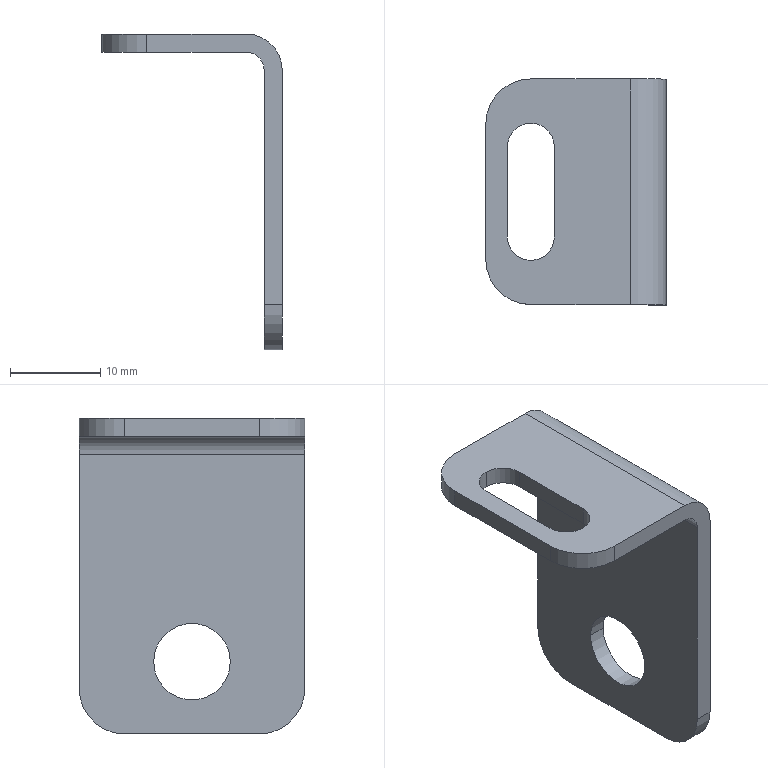Component | SolidWorks | YX-04-119GlueFeedingProximitySwitchFixingPlate-1 | 1 solid | 21 faces | box 20 x 25 x 35 mm | volume 2283 mm3 | cylinder 11 | plane 10 | commonest cylinder face diameters 10 x4 5.2 x3 8.5 x2 4 x1 8 x1 | material SUS340
build123d program:
from build123d import *

# Parameters (mm, degrees)
SKETCH1_W                      = 35
SKETCH1_H                      = 25
BOSS_EXTRUDE1_DEPTH            = 20
SKETCH2_W                      = 33
SKETCH2_H                      = 18
CUT_EXTRUDE1_DEPTH             = 48.434
CUT_EXTRUDE2_DEPTH             = 43.205
F_8_5_8_5_DIAMETER_HOLE1_D     = 8.5
F_8_5_8_5_DIAMETER_HOLE1_DEPTH = 20
FILLET1_R                      = 2
FILLET2_R                      = 4
FILLET3_R                      = 5


with BuildPart() as part:
    # Sketch1 → Boss-Extrude1 (new body)
    with BuildSketch(Plane(origin=(0, 20, 0), x_dir=(1, 0, 0), z_dir=(0, 1, 0))):
        with Locations((17.5, 0)):
            Rectangle(SKETCH1_W, SKETCH1_H)
    extrude(amount=-BOSS_EXTRUDE1_DEPTH)

    # Sketch2 → Cut-Extrude1 (cut, through all)
    with BuildSketch(Plane.XY.offset(12.5)):
        with Locations((18.5, 11)):
            Rectangle(SKETCH2_W, SKETCH2_H)
    extrude(amount=-CUT_EXTRUDE1_DEPTH, mode=Mode.SUBTRACT)

    # Sketch3 → Cut-Extrude2 (cut, through all)
    with BuildSketch(Plane.ZY):
        with BuildLine():
            Line((5, 17.6), (-5, 17.6))
            ThreePointArc((-5, 17.6), (-7.6, 15), (-5, 12.4))
            Line((-5, 12.4), (5, 12.4))
            ThreePointArc((5, 12.4), (7.6, 15), (5, 17.6))
        make_face()
    extrude(amount=-CUT_EXTRUDE2_DEPTH, mode=Mode.SUBTRACT)

    # 8.5 _8.5_ Diameter Hole1
    with Locations(Plane(origin=(0, 0, 0), x_dir=(-1, 0, 0), z_dir=(0, -1, 0))):
        with Locations((-27, 0)):
            Hole(F_8_5_8_5_DIAMETER_HOLE1_D / 2, depth=F_8_5_8_5_DIAMETER_HOLE1_DEPTH)

    # Fillet1
    fillet1_edges = [part.edges().sort_by_distance(p)[0] for p in [
        (2, 2, 0),
    ]]
    fillet(fillet1_edges, radius=FILLET1_R)

    # Fillet2
    fillet2_edges = [part.edges().sort_by_distance(p)[0] for p in [
        (0, 0, 0),
    ]]
    fillet(fillet2_edges, radius=FILLET2_R)

    # Fillet3
    fillet3_edges = [part.edges().sort_by_distance(p)[0] for p in [
        (1, 20, -12.5),
        (1, 20, 12.5),
        (35, 1, -12.5),
        (35, 1, 12.5),
    ]]
    fillet(fillet3_edges, radius=FILLET3_R)


solid = part.part

# Placed as in the assembly
solid = solid.moved(Location((-13.397, 26.962, 194), (-90, 0, 90)))
STEP:
#1=CARTESIAN_POINT('',(-0.6062,1.229,6.575));
#2=VERTEX_POINT('',#1);
#3=CARTESIAN_POINT('',(-0.6062,0.8942,6.575));
#4=VERTEX_POINT('',#3);
#5=CARTESIAN_POINT('',(-0.6062,1.061,6.575));
#6=DIRECTION('',(1.,0.,0.));
#7=DIRECTION('',(0.,-1.,0.));
#8=AXIS2_PLACEMENT_3D('',#5,#6,#7);
#9=CIRCLE('',#8,0.1673);
#10=EDGE_CURVE('',#2,#4,#9,.T.);
#11=ORIENTED_EDGE('',*,*,#10,.F.);
#12=CARTESIAN_POINT('',(-0.5275,1.229,6.575));
#13=VERTEX_POINT('',#12);
#14=CARTESIAN_POINT('',(-0.5275,1.229,6.575));
#15=DIRECTION('',(1.,0.,0.));
#16=VECTOR('',#15,39.37);
#17=LINE('',#14,#16);
#18=EDGE_CURVE('',#2,#13,#17,.T.);
#19=ORIENTED_EDGE('',*,*,#18,.T.);
#20=CARTESIAN_POINT('',(-0.5275,0.8942,6.575));
#21=VERTEX_POINT('',#20);
#22=CARTESIAN_POINT('',(-0.5275,1.061,6.575));
#23=DIRECTION('',(1.,0.,0.));
#24=DIRECTION('',(0.,-1.,0.));
#25=AXIS2_PLACEMENT_3D('',#22,#23,#24);
#26=CIRCLE('',#25,0.1673);
#27=EDGE_CURVE('',#13,#21,#26,.T.);
#28=ORIENTED_EDGE('',*,*,#27,.T.);
#29=CARTESIAN_POINT('',(-0.5275,0.8942,6.575));
#30=DIRECTION('',(1.,0.,0.));
#31=VECTOR('',#30,39.37);
#32=LINE('',#29,#31);
#33=EDGE_CURVE('',#4,#21,#32,.T.);
#34=ORIENTED_EDGE('',*,*,#33,.F.);
#35=EDGE_LOOP('',(#11,#19,#28,#34));
#36=FACE_OUTER_BOUND('',#35,.T.);
#37=CARTESIAN_POINT('',(-0.5275,1.061,6.575));
#38=DIRECTION('',(1.,0.,0.));
#39=DIRECTION('',(0.,-1.,0.));
#40=AXIS2_PLACEMENT_3D('',#37,#38,#39);
#41=CYLINDRICAL_SURFACE('',#40,0.1673);
#42=ADVANCED_FACE('',(#36),#41,.F.);
#43=CARTESIAN_POINT('',(-1.118,1.361,7.559));
#44=VERTEX_POINT('',#43);
#45=CARTESIAN_POINT('',(-1.22,1.258,7.559));
#46=VERTEX_POINT('',#45);
#47=CARTESIAN_POINT('',(-1.118,1.258,7.559));
#48=DIRECTION('',(0.,0.,1.));
#49=DIRECTION('',(1.,0.,0.));
#50=AXIS2_PLACEMENT_3D('',#47,#48,#49);
#51=CIRCLE('',#50,0.1024);
#52=EDGE_CURVE('',#44,#46,#51,.T.);
#53=ORIENTED_EDGE('',*,*,#52,.F.);
#54=CARTESIAN_POINT('',(-1.118,1.361,7.638));
#55=VERTEX_POINT('',#54);
#56=CARTESIAN_POINT('',(-1.118,1.361,6.26));
#57=DIRECTION('',(-0.,0.,1.));
#58=VECTOR('',#57,39.37);
#59=LINE('',#56,#58);
#60=EDGE_CURVE('',#44,#55,#59,.T.);
#61=ORIENTED_EDGE('',*,*,#60,.T.);
#62=CARTESIAN_POINT('',(-1.22,1.258,7.638));
#63=VERTEX_POINT('',#62);
#64=CARTESIAN_POINT('',(-1.118,1.258,7.638));
#65=DIRECTION('',(-0.,0.,1.));
#66=DIRECTION('',(0.,1.,0.));
#67=AXIS2_PLACEMENT_3D('',#64,#65,#66);
#68=CIRCLE('',#67,0.1024);
#69=EDGE_CURVE('',#55,#63,#68,.T.);
#70=ORIENTED_EDGE('',*,*,#69,.T.);
#71=CARTESIAN_POINT('',(-1.22,1.258,6.26));
#72=DIRECTION('',(-0.,0.,1.));
#73=VECTOR('',#72,39.37);
#74=LINE('',#71,#73);
#75=EDGE_CURVE('',#46,#63,#74,.T.);
#76=ORIENTED_EDGE('',*,*,#75,.F.);
#77=EDGE_LOOP('',(#53,#61,#70,#76));
#78=FACE_OUTER_BOUND('',#77,.T.);
#79=CARTESIAN_POINT('',(-1.118,1.258,6.26));
#80=DIRECTION('',(-0.,0.,1.));
#81=DIRECTION('',(0.,1.,0.));
#82=AXIS2_PLACEMENT_3D('',#79,#80,#81);
#83=CYLINDRICAL_SURFACE('',#82,0.1024);
#84=ADVANCED_FACE('',(#78),#83,.F.);
#85=CARTESIAN_POINT('',(-1.016,1.258,7.638));
#86=VERTEX_POINT('',#85);
#87=CARTESIAN_POINT('',(-1.118,1.258,7.638));
#88=DIRECTION('',(-0.,0.,1.));
#89=DIRECTION('',(0.,1.,0.));
#90=AXIS2_PLACEMENT_3D('',#87,#88,#89);
#91=CIRCLE('',#90,0.1024);
#92=EDGE_CURVE('',#86,#55,#91,.T.);
#93=ORIENTED_EDGE('',*,*,#92,.F.);
#94=CARTESIAN_POINT('',(-1.016,0.8646,7.638));
#95=VERTEX_POINT('',#94);
#96=CARTESIAN_POINT('',(-1.016,0.8646,7.638));
#97=DIRECTION('',(-0.,1.,-0.));
#98=VECTOR('',#97,39.37);
#99=LINE('',#96,#98);
#100=EDGE_CURVE('',#95,#86,#99,.T.);
#101=ORIENTED_EDGE('',*,*,#100,.F.);
#102=CARTESIAN_POINT('',(-1.22,0.8646,7.638));
#103=VERTEX_POINT('',#102);
#104=CARTESIAN_POINT('',(-1.118,0.8646,7.638));
#105=DIRECTION('',(-0.,0.,1.));
#106=DIRECTION('',(0.,1.,0.));
#107=AXIS2_PLACEMENT_3D('',#104,#105,#106);
#108=CIRCLE('',#107,0.1024);
#109=EDGE_CURVE('',#103,#95,#108,.T.);
#110=ORIENTED_EDGE('',*,*,#109,.F.);
#111=CARTESIAN_POINT('',(-1.22,1.258,7.638));
#112=DIRECTION('',(0.,-1.,0.));
#113=VECTOR('',#112,39.37);
#114=LINE('',#111,#113);
#115=EDGE_CURVE('',#63,#103,#114,.T.);
#116=ORIENTED_EDGE('',*,*,#115,.F.);
#117=ORIENTED_EDGE('',*,*,#69,.F.);
#118=EDGE_LOOP('',(#93,#101,#110,#116,#117));
#119=FACE_BOUND('',#118,.T.);
#120=CARTESIAN_POINT('',(-1.315,0.7662,7.638));
#121=VERTEX_POINT('',#120);
#122=CARTESIAN_POINT('',(-1.315,1.357,7.638));
#123=VERTEX_POINT('',#122);
#124=CARTESIAN_POINT('',(-1.315,0.5694,7.638));
#125=DIRECTION('',(-0.,1.,-0.));
#126=VECTOR('',#125,39.37);
#127=LINE('',#124,#126);
#128=EDGE_CURVE('',#121,#123,#127,.T.);
#129=ORIENTED_EDGE('',*,*,#128,.F.);
#130=CARTESIAN_POINT('',(-1.118,0.5694,7.638));
#131=VERTEX_POINT('',#130);
#132=CARTESIAN_POINT('',(-1.118,0.7662,7.638));
#133=DIRECTION('',(-0.,0.,1.));
#134=DIRECTION('',(0.,1.,0.));
#135=AXIS2_PLACEMENT_3D('',#132,#133,#134);
#136=CIRCLE('',#135,0.1969);
#137=EDGE_CURVE('',#121,#131,#136,.T.);
#138=ORIENTED_EDGE('',*,*,#137,.T.);
#139=CARTESIAN_POINT('',(-0.6849,0.5694,7.638));
#140=VERTEX_POINT('',#139);
#141=CARTESIAN_POINT('',(-0.5275,0.5694,7.638));
#142=DIRECTION('',(-1.,-0.,-0.));
#143=VECTOR('',#142,39.37);
#144=LINE('',#141,#143);
#145=EDGE_CURVE('',#140,#131,#144,.T.);
#146=ORIENTED_EDGE('',*,*,#145,.F.);
#147=CARTESIAN_POINT('',(-0.6849,1.554,7.638));
#148=VERTEX_POINT('',#147);
#149=CARTESIAN_POINT('',(-0.6849,1.554,7.638));
#150=DIRECTION('',(-0.,1.,-0.));
#151=VECTOR('',#150,39.37);
#152=LINE('',#149,#151);
#153=EDGE_CURVE('',#140,#148,#152,.T.);
#154=ORIENTED_EDGE('',*,*,#153,.T.);
#155=CARTESIAN_POINT('',(-1.118,1.554,7.638));
#156=VERTEX_POINT('',#155);
#157=CARTESIAN_POINT('',(-0.5275,1.554,7.638));
#158=DIRECTION('',(-1.,-0.,-0.));
#159=VECTOR('',#158,39.37);
#160=LINE('',#157,#159);
#161=EDGE_CURVE('',#148,#156,#160,.T.);
#162=ORIENTED_EDGE('',*,*,#161,.T.);
#163=CARTESIAN_POINT('',(-1.118,1.357,7.638));
#164=DIRECTION('',(-0.,0.,1.));
#165=DIRECTION('',(0.,1.,0.));
#166=AXIS2_PLACEMENT_3D('',#163,#164,#165);
#167=CIRCLE('',#166,0.1969);
#168=EDGE_CURVE('',#156,#123,#167,.T.);
#169=ORIENTED_EDGE('',*,*,#168,.T.);
#170=EDGE_LOOP('',(#129,#138,#146,#154,#162,#169));
#171=FACE_OUTER_BOUND('',#170,.T.);
#172=CARTESIAN_POINT('',(-0.5275,0.5694,7.638));
#173=DIRECTION('',(-0.,0.,1.));
#174=DIRECTION('',(-0.,1.,-0.));
#175=AXIS2_PLACEMENT_3D('',#172,#173,#174);
#176=PLANE('',#175);
#177=ADVANCED_FACE('',(#119,#171),#176,.T.);
#178=CARTESIAN_POINT('',(-0.6062,0.5694,7.48));
#179=VERTEX_POINT('',#178);
#180=CARTESIAN_POINT('',(-0.6062,0.5694,6.457));
#181=VERTEX_POINT('',#180);
#182=CARTESIAN_POINT('',(-0.6062,0.5694,7.559));
#183=DIRECTION('',(0.,-0.,-1.));
#184=VECTOR('',#183,39.37);
#185=LINE('',#182,#184);
#186=EDGE_CURVE('',#179,#181,#185,.T.);
#187=ORIENTED_EDGE('',*,*,#186,.T.);
#188=CARTESIAN_POINT('',(-0.5275,0.5694,6.457));
#189=VERTEX_POINT('',#188);
#190=CARTESIAN_POINT('',(-0.5275,0.5694,6.457));
#191=DIRECTION('',(1.,0.,0.));
#192=VECTOR('',#191,39.37);
#193=LINE('',#190,#192);
#194=EDGE_CURVE('',#181,#189,#193,.T.);
#195=ORIENTED_EDGE('',*,*,#194,.T.);
#196=CARTESIAN_POINT('',(-0.5275,0.5694,7.48));
#197=VERTEX_POINT('',#196);
#198=CARTESIAN_POINT('',(-0.5275,0.5694,6.26));
#199=DIRECTION('',(-0.,0.,1.));
#200=VECTOR('',#199,39.37);
#201=LINE('',#198,#200);
#202=EDGE_CURVE('',#189,#197,#201,.T.);
#203=ORIENTED_EDGE('',*,*,#202,.T.);
#204=CARTESIAN_POINT('',(-0.6849,0.5694,7.48));
#205=DIRECTION('',(0.,-1.,0.));
#206=DIRECTION('',(0.,0.,1.));
#207=AXIS2_PLACEMENT_3D('',#204,#205,#206);
#208=CIRCLE('',#207,0.1575);
#209=EDGE_CURVE('',#197,#140,#208,.T.);
#210=ORIENTED_EDGE('',*,*,#209,.T.);
#211=ORIENTED_EDGE('',*,*,#145,.T.);
#212=CARTESIAN_POINT('',(-1.118,0.5694,7.559));
#213=VERTEX_POINT('',#212);
#214=CARTESIAN_POINT('',(-1.118,0.5694,6.26));
#215=DIRECTION('',(0.,-0.,-1.));
#216=VECTOR('',#215,39.37);
#217=LINE('',#214,#216);
#218=EDGE_CURVE('',#131,#213,#217,.T.);
#219=ORIENTED_EDGE('',*,*,#218,.T.);
#220=CARTESIAN_POINT('',(-0.6849,0.5694,7.559));
#221=VERTEX_POINT('',#220);
#222=CARTESIAN_POINT('',(-1.315,0.5694,7.559));
#223=DIRECTION('',(1.,0.,0.));
#224=VECTOR('',#223,39.37);
#225=LINE('',#222,#224);
#226=EDGE_CURVE('',#213,#221,#225,.T.);
#227=ORIENTED_EDGE('',*,*,#226,.T.);
#228=CARTESIAN_POINT('',(-0.6849,0.5694,7.48));
#229=DIRECTION('',(-0.,1.,-0.));
#230=DIRECTION('',(0.,0.,1.));
#231=AXIS2_PLACEMENT_3D('',#228,#229,#230);
#232=CIRCLE('',#231,0.07874);
#233=EDGE_CURVE('',#221,#179,#232,.T.);
#234=ORIENTED_EDGE('',*,*,#233,.T.);
#235=EDGE_LOOP('',(#187,#195,#203,#210,#211,#219,#227,#234));
#236=FACE_OUTER_BOUND('',#235,.T.);
#237=CARTESIAN_POINT('',(-0.5275,0.5694,6.26));
#238=DIRECTION('',(0.,-1.,0.));
#239=DIRECTION('',(-0.,0.,1.));
#240=AXIS2_PLACEMENT_3D('',#237,#238,#239);
#241=PLANE('',#240);
#242=ADVANCED_FACE('',(#236),#241,.T.);
#243=CARTESIAN_POINT('',(-0.5275,1.357,6.26));
#244=VERTEX_POINT('',#243);
#245=CARTESIAN_POINT('',(-0.5275,0.7662,6.26));
#246=VERTEX_POINT('',#245);
#247=CARTESIAN_POINT('',(-0.5275,1.554,6.26));
#248=DIRECTION('',(0.,-1.,0.));
#249=VECTOR('',#248,39.37);
#250=LINE('',#247,#249);
#251=EDGE_CURVE('',#244,#246,#250,.T.);
#252=ORIENTED_EDGE('',*,*,#251,.T.);
#253=CARTESIAN_POINT('',(-0.6062,0.7662,6.26));
#254=VERTEX_POINT('',#253);
#255=CARTESIAN_POINT('',(-0.5275,0.7662,6.26));
#256=DIRECTION('',(-1.,-0.,-0.));
#257=VECTOR('',#256,39.37);
#258=LINE('',#255,#257);
#259=EDGE_CURVE('',#246,#254,#258,.T.);
#260=ORIENTED_EDGE('',*,*,#259,.T.);
#261=CARTESIAN_POINT('',(-0.6062,1.357,6.26));
#262=VERTEX_POINT('',#261);
#263=CARTESIAN_POINT('',(-0.6062,0.5694,6.26));
#264=DIRECTION('',(-0.,1.,-0.));
#265=VECTOR('',#264,39.37);
#266=LINE('',#263,#265);
#267=EDGE_CURVE('',#254,#262,#266,.T.);
#268=ORIENTED_EDGE('',*,*,#267,.T.);
#269=CARTESIAN_POINT('',(-0.5275,1.357,6.26));
#270=DIRECTION('',(1.,0.,0.));
#271=VECTOR('',#270,39.37);
#272=LINE('',#269,#271);
#273=EDGE_CURVE('',#262,#244,#272,.T.);
#274=ORIENTED_EDGE('',*,*,#273,.T.);
#275=EDGE_LOOP('',(#252,#260,#268,#274));
#276=FACE_OUTER_BOUND('',#275,.T.);
#277=CARTESIAN_POINT('',(-0.5275,1.554,6.26));
#278=DIRECTION('',(0.,-0.,-1.));
#279=DIRECTION('',(0.,-1.,0.));
#280=AXIS2_PLACEMENT_3D('',#277,#278,#279);
#281=PLANE('',#280);
#282=ADVANCED_FACE('',(#276),#281,.T.);
#283=CARTESIAN_POINT('',(-0.5275,1.554,7.48));
#284=VERTEX_POINT('',#283);
#285=CARTESIAN_POINT('',(-0.5275,1.554,6.457));
#286=VERTEX_POINT('',#285);
#287=CARTESIAN_POINT('',(-0.5275,1.554,7.638));
#288=DIRECTION('',(0.,-0.,-1.));
#289=VECTOR('',#288,39.37);
#290=LINE('',#287,#289);
#291=EDGE_CURVE('',#284,#286,#290,.T.);
#292=ORIENTED_EDGE('',*,*,#291,.T.);
#293=CARTESIAN_POINT('',(-0.6062,1.554,6.457));
#294=VERTEX_POINT('',#293);
#295=CARTESIAN_POINT('',(-0.5275,1.554,6.457));
#296=DIRECTION('',(-1.,-0.,-0.));
#297=VECTOR('',#296,39.37);
#298=LINE('',#295,#297);
#299=EDGE_CURVE('',#286,#294,#298,.T.);
#300=ORIENTED_EDGE('',*,*,#299,.T.);
#301=CARTESIAN_POINT('',(-0.6062,1.554,7.48));
#302=VERTEX_POINT('',#301);
#303=CARTESIAN_POINT('',(-0.6062,1.554,7.559));
#304=DIRECTION('',(0.,-0.,-1.));
#305=VECTOR('',#304,39.37);
#306=LINE('',#303,#305);
#307=EDGE_CURVE('',#302,#294,#306,.T.);
#308=ORIENTED_EDGE('',*,*,#307,.F.);
#309=CARTESIAN_POINT('',(-0.6849,1.554,7.559));
#310=VERTEX_POINT('',#309);
#311=CARTESIAN_POINT('',(-0.6849,1.554,7.48));
#312=DIRECTION('',(0.,-1.,0.));
#313=DIRECTION('',(0.,0.,-1.));
#314=AXIS2_PLACEMENT_3D('',#311,#312,#313);
#315=CIRCLE('',#314,0.07874);
#316=EDGE_CURVE('',#302,#310,#315,.T.);
#317=ORIENTED_EDGE('',*,*,#316,.T.);
#318=CARTESIAN_POINT('',(-1.118,1.554,7.559));
#319=VERTEX_POINT('',#318);
#320=CARTESIAN_POINT('',(-1.315,1.554,7.559));
#321=DIRECTION('',(1.,0.,0.));
#322=VECTOR('',#321,39.37);
#323=LINE('',#320,#322);
#324=EDGE_CURVE('',#319,#310,#323,.T.);
#325=ORIENTED_EDGE('',*,*,#324,.F.);
#326=CARTESIAN_POINT('',(-1.118,1.554,7.638));
#327=DIRECTION('',(-0.,0.,1.));
#328=VECTOR('',#327,39.37);
#329=LINE('',#326,#328);
#330=EDGE_CURVE('',#319,#156,#329,.T.);
#331=ORIENTED_EDGE('',*,*,#330,.T.);
#332=ORIENTED_EDGE('',*,*,#161,.F.);
#333=CARTESIAN_POINT('',(-0.6849,1.554,7.48));
#334=DIRECTION('',(-0.,1.,-0.));
#335=DIRECTION('',(0.,0.,-1.));
#336=AXIS2_PLACEMENT_3D('',#333,#334,#335);
#337=CIRCLE('',#336,0.1575);
#338=EDGE_CURVE('',#148,#284,#337,.T.);
#339=ORIENTED_EDGE('',*,*,#338,.T.);
#340=EDGE_LOOP('',(#292,#300,#308,#317,#325,#331,#332,#339));
#341=FACE_OUTER_BOUND('',#340,.T.);
#342=CARTESIAN_POINT('',(-0.5275,1.554,7.638));
#343=DIRECTION('',(-0.,1.,-0.));
#344=DIRECTION('',(0.,-0.,-1.));
#345=AXIS2_PLACEMENT_3D('',#342,#343,#344);
#346=PLANE('',#345);
#347=ADVANCED_FACE('',(#341),#346,.T.);
#348=CARTESIAN_POINT('',(-0.5275,1.061,6.575));
#349=DIRECTION('',(1.,0.,0.));
#350=DIRECTION('',(0.,-1.,0.));
#351=AXIS2_PLACEMENT_3D('',#348,#349,#350);
#352=CIRCLE('',#351,0.1673);
#353=EDGE_CURVE('',#21,#13,#352,.T.);
#354=ORIENTED_EDGE('',*,*,#353,.F.);
#355=ORIENTED_EDGE('',*,*,#27,.F.);
#356=EDGE_LOOP('',(#354,#355));
#357=FACE_BOUND('',#356,.T.);
#358=ORIENTED_EDGE('',*,*,#202,.F.);
#359=CARTESIAN_POINT('',(-0.5275,0.7662,6.457));
#360=DIRECTION('',(1.,0.,0.));
#361=DIRECTION('',(0.,1.,0.));
#362=AXIS2_PLACEMENT_3D('',#359,#360,#361);
#363=CIRCLE('',#362,0.1969);
#364=EDGE_CURVE('',#189,#246,#363,.T.);
#365=ORIENTED_EDGE('',*,*,#364,.T.);
#366=ORIENTED_EDGE('',*,*,#251,.F.);
#367=CARTESIAN_POINT('',(-0.5275,1.357,6.457));
#368=DIRECTION('',(1.,0.,0.));
#369=DIRECTION('',(0.,1.,0.));
#370=AXIS2_PLACEMENT_3D('',#367,#368,#369);
#371=CIRCLE('',#370,0.1969);
#372=EDGE_CURVE('',#244,#286,#371,.T.);
#373=ORIENTED_EDGE('',*,*,#372,.T.);
#374=ORIENTED_EDGE('',*,*,#291,.F.);
#375=CARTESIAN_POINT('',(-0.5275,0.5694,7.48));
#376=DIRECTION('',(0.,-1.,0.));
#377=VECTOR('',#376,39.37);
#378=LINE('',#375,#377);
#379=EDGE_CURVE('',#284,#197,#378,.T.);
#380=ORIENTED_EDGE('',*,*,#379,.T.);
#381=EDGE_LOOP('',(#358,#365,#366,#373,#374,#380));
#382=FACE_OUTER_BOUND('',#381,.T.);
#383=CARTESIAN_POINT('',(-0.5275,1.061,7.638));
#384=DIRECTION('',(-1.,-0.,-0.));
#385=DIRECTION('',(-0.,1.,-0.));
#386=AXIS2_PLACEMENT_3D('',#383,#384,#385);
#387=PLANE('',#386);
#388=ADVANCED_FACE('',(#357,#382),#387,.F.);
#389=CARTESIAN_POINT('',(-1.315,0.7662,7.559));
#390=VERTEX_POINT('',#389);
#391=CARTESIAN_POINT('',(-1.315,1.357,7.559));
#392=VERTEX_POINT('',#391);
#393=CARTESIAN_POINT('',(-1.315,0.5694,7.559));
#394=DIRECTION('',(-0.,1.,-0.));
#395=VECTOR('',#394,39.37);
#396=LINE('',#393,#395);
#397=EDGE_CURVE('',#390,#392,#396,.T.);
#398=ORIENTED_EDGE('',*,*,#397,.F.);
#399=CARTESIAN_POINT('',(-1.315,0.7662,7.638));
#400=DIRECTION('',(-0.,0.,1.));
#401=VECTOR('',#400,39.37);
#402=LINE('',#399,#401);
#403=EDGE_CURVE('',#390,#121,#402,.T.);
#404=ORIENTED_EDGE('',*,*,#403,.T.);
#405=ORIENTED_EDGE('',*,*,#128,.T.);
#406=CARTESIAN_POINT('',(-1.315,1.357,7.638));
#407=DIRECTION('',(0.,-0.,-1.));
#408=VECTOR('',#407,39.37);
#409=LINE('',#406,#408);
#410=EDGE_CURVE('',#123,#392,#409,.T.);
#411=ORIENTED_EDGE('',*,*,#410,.T.);
#412=EDGE_LOOP('',(#398,#404,#405,#411));
#413=FACE_OUTER_BOUND('',#412,.T.);
#414=CARTESIAN_POINT('',(-1.315,1.061,7.638));
#415=DIRECTION('',(-1.,-0.,-0.));
#416=DIRECTION('',(-0.,1.,-0.));
#417=AXIS2_PLACEMENT_3D('',#414,#415,#416);
#418=PLANE('',#417);
#419=ADVANCED_FACE('',(#413),#418,.T.);
#420=CARTESIAN_POINT('',(-0.6062,1.061,6.575));
#421=DIRECTION('',(1.,0.,0.));
#422=DIRECTION('',(0.,-1.,0.));
#423=AXIS2_PLACEMENT_3D('',#420,#421,#422);
#424=CIRCLE('',#423,0.1673);
#425=EDGE_CURVE('',#4,#2,#424,.T.);
#426=ORIENTED_EDGE('',*,*,#425,.T.);
#427=ORIENTED_EDGE('',*,*,#10,.T.);
#428=EDGE_LOOP('',(#426,#427));
#429=FACE_BOUND('',#428,.T.);
#430=ORIENTED_EDGE('',*,*,#267,.F.);
#431=CARTESIAN_POINT('',(-0.6062,0.7662,6.457));
#432=DIRECTION('',(-1.,-0.,-0.));
#433=DIRECTION('',(0.,-1.,0.));
#434=AXIS2_PLACEMENT_3D('',#431,#432,#433);
#435=CIRCLE('',#434,0.1969);
#436=EDGE_CURVE('',#254,#181,#435,.T.);
#437=ORIENTED_EDGE('',*,*,#436,.T.);
#438=ORIENTED_EDGE('',*,*,#186,.F.);
#439=CARTESIAN_POINT('',(-0.6062,1.554,7.48));
#440=DIRECTION('',(-0.,1.,-0.));
#441=VECTOR('',#440,39.37);
#442=LINE('',#439,#441);
#443=EDGE_CURVE('',#179,#302,#442,.T.);
#444=ORIENTED_EDGE('',*,*,#443,.T.);
#445=ORIENTED_EDGE('',*,*,#307,.T.);
#446=CARTESIAN_POINT('',(-0.6062,1.357,6.457));
#447=DIRECTION('',(-1.,-0.,-0.));
#448=DIRECTION('',(0.,-1.,0.));
#449=AXIS2_PLACEMENT_3D('',#446,#447,#448);
#450=CIRCLE('',#449,0.1969);
#451=EDGE_CURVE('',#294,#262,#450,.T.);
#452=ORIENTED_EDGE('',*,*,#451,.T.);
#453=EDGE_LOOP('',(#430,#437,#438,#444,#445,#452));
#454=FACE_OUTER_BOUND('',#453,.T.);
#455=CARTESIAN_POINT('',(-0.6062,0.5694,7.559));
#456=DIRECTION('',(1.,0.,0.));
#457=DIRECTION('',(0.,-1.,0.));
#458=AXIS2_PLACEMENT_3D('',#455,#456,#457);
#459=PLANE('',#458);
#460=ADVANCED_FACE('',(#429,#454),#459,.F.);
#461=CARTESIAN_POINT('',(-1.016,0.8646,7.559));
#462=VERTEX_POINT('',#461);
#463=CARTESIAN_POINT('',(-1.016,1.258,7.559));
#464=VERTEX_POINT('',#463);
#465=CARTESIAN_POINT('',(-1.016,0.5694,7.559));
#466=DIRECTION('',(-0.,1.,-0.));
#467=VECTOR('',#466,39.37);
#468=LINE('',#465,#467);
#469=EDGE_CURVE('',#462,#464,#468,.T.);
#470=ORIENTED_EDGE('',*,*,#469,.T.);
#471=CARTESIAN_POINT('',(-1.118,1.258,7.559));
#472=DIRECTION('',(0.,0.,1.));
#473=DIRECTION('',(1.,0.,0.));
#474=AXIS2_PLACEMENT_3D('',#471,#472,#473);
#475=CIRCLE('',#474,0.1024);
#476=EDGE_CURVE('',#464,#44,#475,.T.);
#477=ORIENTED_EDGE('',*,*,#476,.T.);
#478=ORIENTED_EDGE('',*,*,#52,.T.);
#479=CARTESIAN_POINT('',(-1.22,0.8646,7.559));
#480=VERTEX_POINT('',#479);
#481=CARTESIAN_POINT('',(-1.22,0.5694,7.559));
#482=DIRECTION('',(0.,-1.,0.));
#483=VECTOR('',#482,39.37);
#484=LINE('',#481,#483);
#485=EDGE_CURVE('',#46,#480,#484,.T.);
#486=ORIENTED_EDGE('',*,*,#485,.T.);
#487=CARTESIAN_POINT('',(-1.118,0.8646,7.559));
#488=DIRECTION('',(0.,0.,1.));
#489=DIRECTION('',(1.,0.,0.));
#490=AXIS2_PLACEMENT_3D('',#487,#488,#489);
#491=CIRCLE('',#490,0.1024);
#492=EDGE_CURVE('',#480,#462,#491,.T.);
#493=ORIENTED_EDGE('',*,*,#492,.T.);
#494=EDGE_LOOP('',(#470,#477,#478,#486,#493));
#495=FACE_BOUND('',#494,.T.);
#496=ORIENTED_EDGE('',*,*,#226,.F.);
#497=CARTESIAN_POINT('',(-1.118,0.7662,7.559));
#498=DIRECTION('',(-0.,-0.,-1.));
#499=DIRECTION('',(1.,0.,0.));
#500=AXIS2_PLACEMENT_3D('',#497,#498,#499);
#501=CIRCLE('',#500,0.1969);
#502=EDGE_CURVE('',#213,#390,#501,.T.);
#503=ORIENTED_EDGE('',*,*,#502,.T.);
#504=ORIENTED_EDGE('',*,*,#397,.T.);
#505=CARTESIAN_POINT('',(-1.118,1.357,7.559));
#506=DIRECTION('',(-0.,-0.,-1.));
#507=DIRECTION('',(1.,0.,0.));
#508=AXIS2_PLACEMENT_3D('',#505,#506,#507);
#509=CIRCLE('',#508,0.1969);
#510=EDGE_CURVE('',#392,#319,#509,.T.);
#511=ORIENTED_EDGE('',*,*,#510,.T.);
#512=ORIENTED_EDGE('',*,*,#324,.T.);
#513=CARTESIAN_POINT('',(-0.6849,0.5694,7.559));
#514=DIRECTION('',(0.,-1.,0.));
#515=VECTOR('',#514,39.37);
#516=LINE('',#513,#515);
#517=EDGE_CURVE('',#310,#221,#516,.T.);
#518=ORIENTED_EDGE('',*,*,#517,.T.);
#519=EDGE_LOOP('',(#496,#503,#504,#511,#512,#518));
#520=FACE_OUTER_BOUND('',#519,.T.);
#521=CARTESIAN_POINT('',(-1.315,0.5694,7.559));
#522=DIRECTION('',(-0.,0.,1.));
#523=DIRECTION('',(1.,0.,0.));
#524=AXIS2_PLACEMENT_3D('',#521,#522,#523);
#525=PLANE('',#524);
#526=ADVANCED_FACE('',(#495,#520),#525,.F.);
#527=ORIENTED_EDGE('',*,*,#60,.F.);
#528=ORIENTED_EDGE('',*,*,#476,.F.);
#529=CARTESIAN_POINT('',(-1.016,1.258,6.26));
#530=DIRECTION('',(-0.,0.,1.));
#531=VECTOR('',#530,39.37);
#532=LINE('',#529,#531);
#533=EDGE_CURVE('',#464,#86,#532,.T.);
#534=ORIENTED_EDGE('',*,*,#533,.T.);
#535=ORIENTED_EDGE('',*,*,#92,.T.);
#536=EDGE_LOOP('',(#527,#528,#534,#535));
#537=FACE_OUTER_BOUND('',#536,.T.);
#538=CARTESIAN_POINT('',(-1.118,1.258,6.26));
#539=DIRECTION('',(-0.,0.,1.));
#540=DIRECTION('',(0.,1.,0.));
#541=AXIS2_PLACEMENT_3D('',#538,#539,#540);
#542=CYLINDRICAL_SURFACE('',#541,0.1024);
#543=ADVANCED_FACE('',(#537),#542,.F.);
#544=CARTESIAN_POINT('',(-1.016,0.8646,6.26));
#545=DIRECTION('',(-0.,0.,1.));
#546=VECTOR('',#545,39.37);
#547=LINE('',#544,#546);
#548=EDGE_CURVE('',#462,#95,#547,.T.);
#549=ORIENTED_EDGE('',*,*,#548,.T.);
#550=ORIENTED_EDGE('',*,*,#100,.T.);
#551=ORIENTED_EDGE('',*,*,#533,.F.);
#552=ORIENTED_EDGE('',*,*,#469,.F.);
#553=EDGE_LOOP('',(#549,#550,#551,#552));
#554=FACE_OUTER_BOUND('',#553,.T.);
#555=CARTESIAN_POINT('',(-1.016,0.8646,6.26));
#556=DIRECTION('',(1.,0.,0.));
#557=DIRECTION('',(0.,-1.,0.));
#558=AXIS2_PLACEMENT_3D('',#555,#556,#557);
#559=PLANE('',#558);
#560=ADVANCED_FACE('',(#554),#559,.F.);
#561=CARTESIAN_POINT('',(-1.22,0.8646,6.26));
#562=DIRECTION('',(-0.,0.,1.));
#563=VECTOR('',#562,39.37);
#564=LINE('',#561,#563);
#565=EDGE_CURVE('',#480,#103,#564,.T.);
#566=ORIENTED_EDGE('',*,*,#565,.T.);
#567=ORIENTED_EDGE('',*,*,#109,.T.);
#568=ORIENTED_EDGE('',*,*,#548,.F.);
#569=ORIENTED_EDGE('',*,*,#492,.F.);
#570=EDGE_LOOP('',(#566,#567,#568,#569));
#571=FACE_OUTER_BOUND('',#570,.T.);
#572=CARTESIAN_POINT('',(-1.118,0.8646,6.26));
#573=DIRECTION('',(-0.,0.,1.));
#574=DIRECTION('',(0.,1.,0.));
#575=AXIS2_PLACEMENT_3D('',#572,#573,#574);
#576=CYLINDRICAL_SURFACE('',#575,0.1024);
#577=ADVANCED_FACE('',(#571),#576,.F.);
#578=ORIENTED_EDGE('',*,*,#75,.T.);
#579=ORIENTED_EDGE('',*,*,#115,.T.);
#580=ORIENTED_EDGE('',*,*,#565,.F.);
#581=ORIENTED_EDGE('',*,*,#485,.F.);
#582=EDGE_LOOP('',(#578,#579,#580,#581));
#583=FACE_OUTER_BOUND('',#582,.T.);
#584=CARTESIAN_POINT('',(-1.22,1.258,6.26));
#585=DIRECTION('',(-1.,-0.,-0.));
#586=DIRECTION('',(-0.,1.,-0.));
#587=AXIS2_PLACEMENT_3D('',#584,#585,#586);
#588=PLANE('',#587);
#589=ADVANCED_FACE('',(#583),#588,.F.);
#590=ORIENTED_EDGE('',*,*,#18,.F.);
#591=ORIENTED_EDGE('',*,*,#425,.F.);
#592=ORIENTED_EDGE('',*,*,#33,.T.);
#593=ORIENTED_EDGE('',*,*,#353,.T.);
#594=EDGE_LOOP('',(#590,#591,#592,#593));
#595=FACE_OUTER_BOUND('',#594,.T.);
#596=CARTESIAN_POINT('',(-0.5275,1.061,6.575));
#597=DIRECTION('',(1.,0.,0.));
#598=DIRECTION('',(0.,-1.,0.));
#599=AXIS2_PLACEMENT_3D('',#596,#597,#598);
#600=CYLINDRICAL_SURFACE('',#599,0.1673);
#601=ADVANCED_FACE('',(#595),#600,.F.);
#602=ORIENTED_EDGE('',*,*,#233,.F.);
#603=ORIENTED_EDGE('',*,*,#517,.F.);
#604=ORIENTED_EDGE('',*,*,#316,.F.);
#605=ORIENTED_EDGE('',*,*,#443,.F.);
#606=EDGE_LOOP('',(#602,#603,#604,#605));
#607=FACE_OUTER_BOUND('',#606,.T.);
#608=CARTESIAN_POINT('',(-0.6849,0.5694,7.48));
#609=DIRECTION('',(0.,-1.,0.));
#610=DIRECTION('',(0.,0.,1.));
#611=AXIS2_PLACEMENT_3D('',#608,#609,#610);
#612=CYLINDRICAL_SURFACE('',#611,0.07874);
#613=ADVANCED_FACE('',(#607),#612,.F.);
#614=ORIENTED_EDGE('',*,*,#209,.F.);
#615=ORIENTED_EDGE('',*,*,#379,.F.);
#616=ORIENTED_EDGE('',*,*,#338,.F.);
#617=ORIENTED_EDGE('',*,*,#153,.F.);
#618=EDGE_LOOP('',(#614,#615,#616,#617));
#619=FACE_OUTER_BOUND('',#618,.T.);
#620=CARTESIAN_POINT('',(-0.6849,0.5694,7.48));
#621=DIRECTION('',(0.,-1.,0.));
#622=DIRECTION('',(0.,0.,1.));
#623=AXIS2_PLACEMENT_3D('',#620,#621,#622);
#624=CYLINDRICAL_SURFACE('',#623,0.1575);
#625=ADVANCED_FACE('',(#619),#624,.T.);
#626=ORIENTED_EDGE('',*,*,#364,.F.);
#627=ORIENTED_EDGE('',*,*,#194,.F.);
#628=ORIENTED_EDGE('',*,*,#436,.F.);
#629=ORIENTED_EDGE('',*,*,#259,.F.);
#630=EDGE_LOOP('',(#626,#627,#628,#629));
#631=FACE_OUTER_BOUND('',#630,.T.);
#632=CARTESIAN_POINT('',(-0.5275,0.7662,6.457));
#633=DIRECTION('',(-1.,-0.,-0.));
#634=DIRECTION('',(0.,1.,0.));
#635=AXIS2_PLACEMENT_3D('',#632,#633,#634);
#636=CYLINDRICAL_SURFACE('',#635,0.1969);
#637=ADVANCED_FACE('',(#631),#636,.T.);
#638=ORIENTED_EDGE('',*,*,#502,.F.);
#639=ORIENTED_EDGE('',*,*,#218,.F.);
#640=ORIENTED_EDGE('',*,*,#137,.F.);
#641=ORIENTED_EDGE('',*,*,#403,.F.);
#642=EDGE_LOOP('',(#638,#639,#640,#641));
#643=FACE_OUTER_BOUND('',#642,.T.);
#644=CARTESIAN_POINT('',(-1.118,0.7662,7.638));
#645=DIRECTION('',(-0.,0.,1.));
#646=DIRECTION('',(0.,1.,0.));
#647=AXIS2_PLACEMENT_3D('',#644,#645,#646);
#648=CYLINDRICAL_SURFACE('',#647,0.1969);
#649=ADVANCED_FACE('',(#643),#648,.T.);
#650=ORIENTED_EDGE('',*,*,#372,.F.);
#651=ORIENTED_EDGE('',*,*,#273,.F.);
#652=ORIENTED_EDGE('',*,*,#451,.F.);
#653=ORIENTED_EDGE('',*,*,#299,.F.);
#654=EDGE_LOOP('',(#650,#651,#652,#653));
#655=FACE_OUTER_BOUND('',#654,.T.);
#656=CARTESIAN_POINT('',(-0.5275,1.357,6.457));
#657=DIRECTION('',(-1.,-0.,-0.));
#658=DIRECTION('',(0.,1.,0.));
#659=AXIS2_PLACEMENT_3D('',#656,#657,#658);
#660=CYLINDRICAL_SURFACE('',#659,0.1969);
#661=ADVANCED_FACE('',(#655),#660,.T.);
#662=ORIENTED_EDGE('',*,*,#168,.F.);
#663=ORIENTED_EDGE('',*,*,#330,.F.);
#664=ORIENTED_EDGE('',*,*,#510,.F.);
#665=ORIENTED_EDGE('',*,*,#410,.F.);
#666=EDGE_LOOP('',(#662,#663,#664,#665));
#667=FACE_OUTER_BOUND('',#666,.T.);
#668=CARTESIAN_POINT('',(-1.118,1.357,7.638));
#669=DIRECTION('',(0.,-0.,-1.));
#670=DIRECTION('',(0.,-1.,0.));
#671=AXIS2_PLACEMENT_3D('',#668,#669,#670);
#672=CYLINDRICAL_SURFACE('',#671,0.1969);
#673=ADVANCED_FACE('',(#667),#672,.T.);
#674=CLOSED_SHELL('',(#42,#84,#177,#242,#282,#347,#388,#419,#460,#526,#543,#560,#577,#589,#601,#613,#625,#637,#649,#661,#673));
#675=MANIFOLD_SOLID_BREP('',#674);
#676=CARTESIAN_POINT('',(0.,0.,0.));
#677=DIRECTION('',(0.,0.,1.));
#678=DIRECTION('',(1.,0.,0.));
#679=AXIS2_PLACEMENT_3D('',#676,#677,#678);
#680=(LENGTH_UNIT()NAMED_UNIT(*)SI_UNIT($,.METRE.));
#681=LENGTH_MEASURE_WITH_UNIT(LENGTH_MEASURE(0.0254),#680);
#682=DIMENSIONAL_EXPONENTS(1.,0.,0.,0.,0.,0.,0.);
#683=(CONVERSION_BASED_UNIT('',#681)LENGTH_UNIT()NAMED_UNIT(#682));
#684=UNCERTAINTY_MEASURE_WITH_UNIT(LENGTH_MEASURE(0.00001),#683,'','');
#685=(NAMED_UNIT(*)PLANE_ANGLE_UNIT()SI_UNIT($,.RADIAN.));
#686=(NAMED_UNIT(*)SI_UNIT($,.STERADIAN.)SOLID_ANGLE_UNIT());
#687=(GEOMETRIC_REPRESENTATION_CONTEXT(3)GLOBAL_UNCERTAINTY_ASSIGNED_CONTEXT((#684))GLOBAL_UNIT_ASSIGNED_CONTEXT((#683,#685,#686))REPRESENTATION_CONTEXT('',''));
#688=ADVANCED_BREP_SHAPE_REPRESENTATION('',(#675,#679),#687);
#689=COLOUR_RGB('',0.7922,0.8196,0.9333);
#690=FILL_AREA_STYLE_COLOUR('',#689);
#691=FILL_AREA_STYLE('',(#690));
#692=SURFACE_STYLE_FILL_AREA(#691);
#693=SURFACE_SIDE_STYLE('',(#692));
#694=SURFACE_STYLE_USAGE(.BOTH.,#693);
#695=PRESENTATION_STYLE_ASSIGNMENT((#694));
#696=STYLED_ITEM('',(#695),#675);
#697=(LENGTH_UNIT()NAMED_UNIT(*)SI_UNIT($,.METRE.));
#698=LENGTH_MEASURE_WITH_UNIT(LENGTH_MEASURE(0.0254),#697);
#699=DIMENSIONAL_EXPONENTS(1.,0.,0.,0.,0.,0.,0.);
#700=(CONVERSION_BASED_UNIT('',#698)LENGTH_UNIT()NAMED_UNIT(#699));
#701=UNCERTAINTY_MEASURE_WITH_UNIT(LENGTH_MEASURE(0.00001),#700,'','');
#702=(NAMED_UNIT(*)PLANE_ANGLE_UNIT()SI_UNIT($,.RADIAN.));
#703=(NAMED_UNIT(*)SI_UNIT($,.STERADIAN.)SOLID_ANGLE_UNIT());
#704=(GEOMETRIC_REPRESENTATION_CONTEXT(3)GLOBAL_UNCERTAINTY_ASSIGNED_CONTEXT((#701))GLOBAL_UNIT_ASSIGNED_CONTEXT((#700,#702,#703))REPRESENTATION_CONTEXT('',''));
#705=MECHANICAL_DESIGN_GEOMETRIC_PRESENTATION_REPRESENTATION('',(#696),#704);
#706=PRESENTATION_LAYER_ASSIGNMENT('','',(#696));